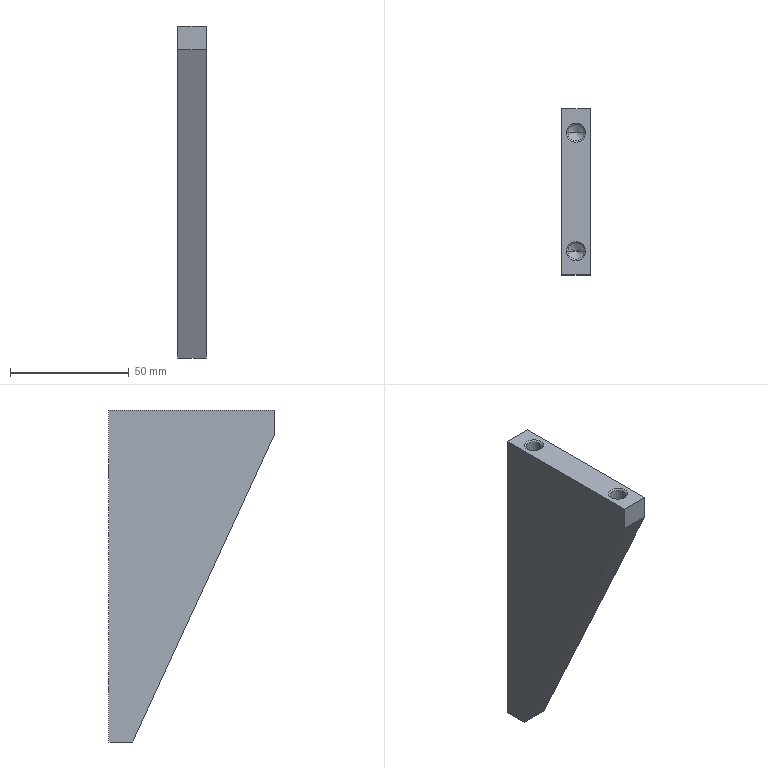Component | SolidWorks | DoubleFilmTransport-1_FilmPullingFixingBaseSupportPlate-2 | 1 solid | 31 faces | box 12 x 70 x 140 mm | volume 68032 mm3 | cone 16 | cylinder 8 | plane 7 | commonest cylinder face diameters 6.8 x8
build123d program:
from build123d import *

# Parameters (mm, degrees)
BOSS_EXTRUDE1_DEPTH            = 12
F_6_8_6_8_DIAMETER_HOLE1_D     = 6.8
F_6_8_6_8_DIAMETER_HOLE1_DEPTH = 18.25
F_6_8_6_8_DIAMETER_HOLE1_TIP   = 2.043
F_6_8_6_8_DIAMETER_HOLE2_D     = 6.8
F_6_8_6_8_DIAMETER_HOLE2_DEPTH = 18.25
F_6_8_6_8_DIAMETER_HOLE2_TIP   = 2.043
CHAMFER1_SIZE                  = 0.625


with BuildPart() as part:
    # Sketch1 → Boss-Extrude1 (new body)
    with BuildSketch(Plane(origin=(0, 0, -6), x_dir=(-1, 0, 0), z_dir=(0, 0, -1))):
        Polygon((0, 0), (0, 140), (-10, 140), (-70, 10), (-70, 0), align=None)
    extrude(amount=-BOSS_EXTRUDE1_DEPTH)

    # 6.8 _6.8_ Diameter Hole1
    with Locations(Plane.ZY):
        with Locations((0, 115), (0, 25)):
            Hole(F_6_8_6_8_DIAMETER_HOLE1_D / 2, depth=F_6_8_6_8_DIAMETER_HOLE1_DEPTH)
            with Locations((0, 0, -(F_6_8_6_8_DIAMETER_HOLE1_DEPTH + F_6_8_6_8_DIAMETER_HOLE1_TIP / 2))):  # 118° drill point
                Cone(0, F_6_8_6_8_DIAMETER_HOLE1_D / 2, F_6_8_6_8_DIAMETER_HOLE1_TIP, mode=Mode.SUBTRACT)

    # 6.8 _6.8_ Diameter Hole2
    with Locations(Plane(origin=(0, 0, 0), x_dir=(-1, 0, 0), z_dir=(0, -1, 0))):
        with Locations((-60, 0), (-10, 0)):
            Hole(F_6_8_6_8_DIAMETER_HOLE2_D / 2, depth=F_6_8_6_8_DIAMETER_HOLE2_DEPTH)
            with Locations((0, 0, -(F_6_8_6_8_DIAMETER_HOLE2_DEPTH + F_6_8_6_8_DIAMETER_HOLE2_TIP / 2))):  # 118° drill point
                Cone(0, F_6_8_6_8_DIAMETER_HOLE2_D / 2, F_6_8_6_8_DIAMETER_HOLE2_TIP, mode=Mode.SUBTRACT)

    # Chamfer1
    chamfer1_edges = [part.edges().sort_by_distance(p)[0] for p in [
        (0, 25, 3.4),
        (0, 115, 3.4),
        (6.6, 0, 0),
        (56.6, 0, 0),
    ]]
    chamfer(chamfer1_edges, length=CHAMFER1_SIZE)


solid = part.part

# Placed as in the assembly
solid = solid.moved(Location((-438.746, 33.373, -31.5), (-90, 90, 0)))
STEP:
#1=COLOUR_RGB('',0.7922,0.8196,0.9333);
#2=FILL_AREA_STYLE_COLOUR('',#1);
#3=FILL_AREA_STYLE('',(#2));
#4=SURFACE_STYLE_FILL_AREA(#3);
#5=SURFACE_SIDE_STYLE('',(#4));
#6=SURFACE_STYLE_USAGE(.BOTH.,#5);
#7=PRESENTATION_STYLE_ASSIGNMENT((#6));
#8=CARTESIAN_POINT('',(-17.14,0.9202,-1.265));
#9=VERTEX_POINT('',#8);
#10=CARTESIAN_POINT('',(-17.407,0.9202,-1.265));
#11=VERTEX_POINT('',#10);
#12=CARTESIAN_POINT('',(-17.273,0.9202,-1.265));
#13=DIRECTION('',(0.,0.,1.));
#14=DIRECTION('',(-1.,0.,0.));
#15=AXIS2_PLACEMENT_3D('',#12,#13,#14);
#16=CIRCLE('',#15,0.1339);
#17=EDGE_CURVE('',#9,#11,#16,.T.);
#18=ORIENTED_EDGE('',*,*,#17,.F.);
#19=CARTESIAN_POINT('',(-17.115,0.9202,-1.24));
#20=VERTEX_POINT('',#19);
#21=CARTESIAN_POINT('',(-17.14,0.9202,-1.265));
#22=DIRECTION('',(0.7071,0.,0.7071));
#23=VECTOR('',#22,39.37);
#24=LINE('',#21,#23);
#25=EDGE_CURVE('',#9,#20,#24,.T.);
#26=ORIENTED_EDGE('',*,*,#25,.T.);
#27=CARTESIAN_POINT('',(-17.432,0.9202,-1.24));
#28=VERTEX_POINT('',#27);
#29=CARTESIAN_POINT('',(-17.273,0.9202,-1.24));
#30=DIRECTION('',(-0.,0.,-1.));
#31=DIRECTION('',(0.,-1.,0.));
#32=AXIS2_PLACEMENT_3D('',#29,#30,#31);
#33=CIRCLE('',#32,0.1585);
#34=EDGE_CURVE('',#28,#20,#33,.T.);
#35=ORIENTED_EDGE('',*,*,#34,.F.);
#36=CARTESIAN_POINT('',(-17.407,0.9202,-1.265));
#37=DIRECTION('',(-0.7071,-0.,0.7071));
#38=VECTOR('',#37,39.37);
#39=LINE('',#36,#38);
#40=EDGE_CURVE('',#11,#28,#39,.T.);
#41=ORIENTED_EDGE('',*,*,#40,.F.);
#42=EDGE_LOOP('',(#18,#26,#35,#41));
#43=FACE_OUTER_BOUND('',#42,.T.);
#44=CARTESIAN_POINT('',(-17.273,0.9202,-1.265));
#45=DIRECTION('',(0.,0.,1.));
#46=DIRECTION('',(-1.,0.,0.));
#47=AXIS2_PLACEMENT_3D('',#44,#45,#46);
#48=CONICAL_SURFACE('',#47,0.1339,0.7854);
#49=ADVANCED_FACE('',(#43),#48,.F.);
#50=CARTESIAN_POINT('',(-17.14,-1.048,-1.265));
#51=VERTEX_POINT('',#50);
#52=CARTESIAN_POINT('',(-17.407,-1.048,-1.265));
#53=VERTEX_POINT('',#52);
#54=CARTESIAN_POINT('',(-17.273,-1.048,-1.265));
#55=DIRECTION('',(0.,0.,1.));
#56=DIRECTION('',(-1.,0.,0.));
#57=AXIS2_PLACEMENT_3D('',#54,#55,#56);
#58=CIRCLE('',#57,0.1339);
#59=EDGE_CURVE('',#51,#53,#58,.T.);
#60=ORIENTED_EDGE('',*,*,#59,.F.);
#61=CARTESIAN_POINT('',(-17.115,-1.048,-1.24));
#62=VERTEX_POINT('',#61);
#63=CARTESIAN_POINT('',(-17.14,-1.048,-1.265));
#64=DIRECTION('',(0.7071,0.,0.7071));
#65=VECTOR('',#64,39.37);
#66=LINE('',#63,#65);
#67=EDGE_CURVE('',#51,#62,#66,.T.);
#68=ORIENTED_EDGE('',*,*,#67,.T.);
#69=CARTESIAN_POINT('',(-17.432,-1.048,-1.24));
#70=VERTEX_POINT('',#69);
#71=CARTESIAN_POINT('',(-17.273,-1.048,-1.24));
#72=DIRECTION('',(-0.,0.,-1.));
#73=DIRECTION('',(0.,-1.,0.));
#74=AXIS2_PLACEMENT_3D('',#71,#72,#73);
#75=CIRCLE('',#74,0.1585);
#76=EDGE_CURVE('',#70,#62,#75,.T.);
#77=ORIENTED_EDGE('',*,*,#76,.F.);
#78=CARTESIAN_POINT('',(-17.407,-1.048,-1.265));
#79=DIRECTION('',(-0.7071,-0.,0.7071));
#80=VECTOR('',#79,39.37);
#81=LINE('',#78,#80);
#82=EDGE_CURVE('',#53,#70,#81,.T.);
#83=ORIENTED_EDGE('',*,*,#82,.F.);
#84=EDGE_LOOP('',(#60,#68,#77,#83));
#85=FACE_OUTER_BOUND('',#84,.T.);
#86=CARTESIAN_POINT('',(-17.273,-1.048,-1.265));
#87=DIRECTION('',(0.,0.,1.));
#88=DIRECTION('',(-1.,0.,0.));
#89=AXIS2_PLACEMENT_3D('',#86,#87,#88);
#90=CONICAL_SURFACE('',#89,0.1339,0.7854);
#91=ADVANCED_FACE('',(#85),#90,.F.);
#92=CARTESIAN_POINT('',(-17.407,1.289,-5.768));
#93=VERTEX_POINT('',#92);
#94=CARTESIAN_POINT('',(-17.14,1.289,-5.768));
#95=VERTEX_POINT('',#94);
#96=CARTESIAN_POINT('',(-17.273,1.289,-5.768));
#97=DIRECTION('',(-0.,1.,0.));
#98=DIRECTION('',(1.,0.,0.));
#99=AXIS2_PLACEMENT_3D('',#96,#97,#98);
#100=CIRCLE('',#99,0.1339);
#101=EDGE_CURVE('',#93,#95,#100,.T.);
#102=ORIENTED_EDGE('',*,*,#101,.F.);
#103=CARTESIAN_POINT('',(-17.432,1.314,-5.768));
#104=VERTEX_POINT('',#103);
#105=CARTESIAN_POINT('',(-17.407,1.289,-5.768));
#106=DIRECTION('',(-0.7071,0.7071,-0.));
#107=VECTOR('',#106,39.37);
#108=LINE('',#105,#107);
#109=EDGE_CURVE('',#93,#104,#108,.T.);
#110=ORIENTED_EDGE('',*,*,#109,.T.);
#111=CARTESIAN_POINT('',(-17.115,1.314,-5.768));
#112=VERTEX_POINT('',#111);
#113=CARTESIAN_POINT('',(-17.273,1.314,-5.768));
#114=DIRECTION('',(0.,-1.,0.));
#115=DIRECTION('',(1.,0.,0.));
#116=AXIS2_PLACEMENT_3D('',#113,#114,#115);
#117=CIRCLE('',#116,0.1585);
#118=EDGE_CURVE('',#112,#104,#117,.T.);
#119=ORIENTED_EDGE('',*,*,#118,.F.);
#120=CARTESIAN_POINT('',(-17.14,1.289,-5.768));
#121=DIRECTION('',(0.7071,0.7071,0.));
#122=VECTOR('',#121,39.37);
#123=LINE('',#120,#122);
#124=EDGE_CURVE('',#95,#112,#123,.T.);
#125=ORIENTED_EDGE('',*,*,#124,.F.);
#126=EDGE_LOOP('',(#102,#110,#119,#125));
#127=FACE_OUTER_BOUND('',#126,.T.);
#128=CARTESIAN_POINT('',(-17.273,1.289,-5.768));
#129=DIRECTION('',(-0.,1.,0.));
#130=DIRECTION('',(1.,0.,0.));
#131=AXIS2_PLACEMENT_3D('',#128,#129,#130);
#132=CONICAL_SURFACE('',#131,0.1339,0.7854);
#133=ADVANCED_FACE('',(#127),#132,.F.);
#134=CARTESIAN_POINT('',(-17.407,1.289,-2.224));
#135=VERTEX_POINT('',#134);
#136=CARTESIAN_POINT('',(-17.14,1.289,-2.224));
#137=VERTEX_POINT('',#136);
#138=CARTESIAN_POINT('',(-17.273,1.289,-2.224));
#139=DIRECTION('',(-0.,1.,0.));
#140=DIRECTION('',(1.,0.,0.));
#141=AXIS2_PLACEMENT_3D('',#138,#139,#140);
#142=CIRCLE('',#141,0.1339);
#143=EDGE_CURVE('',#135,#137,#142,.T.);
#144=ORIENTED_EDGE('',*,*,#143,.F.);
#145=CARTESIAN_POINT('',(-17.432,1.314,-2.224));
#146=VERTEX_POINT('',#145);
#147=CARTESIAN_POINT('',(-17.407,1.289,-2.224));
#148=DIRECTION('',(-0.7071,0.7071,-0.));
#149=VECTOR('',#148,39.37);
#150=LINE('',#147,#149);
#151=EDGE_CURVE('',#135,#146,#150,.T.);
#152=ORIENTED_EDGE('',*,*,#151,.T.);
#153=CARTESIAN_POINT('',(-17.115,1.314,-2.224));
#154=VERTEX_POINT('',#153);
#155=CARTESIAN_POINT('',(-17.273,1.314,-2.224));
#156=DIRECTION('',(0.,-1.,0.));
#157=DIRECTION('',(1.,0.,0.));
#158=AXIS2_PLACEMENT_3D('',#155,#156,#157);
#159=CIRCLE('',#158,0.1585);
#160=EDGE_CURVE('',#154,#146,#159,.T.);
#161=ORIENTED_EDGE('',*,*,#160,.F.);
#162=CARTESIAN_POINT('',(-17.14,1.289,-2.224));
#163=DIRECTION('',(0.7071,0.7071,0.));
#164=VECTOR('',#163,39.37);
#165=LINE('',#162,#164);
#166=EDGE_CURVE('',#137,#154,#165,.T.);
#167=ORIENTED_EDGE('',*,*,#166,.F.);
#168=EDGE_LOOP('',(#144,#152,#161,#167));
#169=FACE_OUTER_BOUND('',#168,.T.);
#170=CARTESIAN_POINT('',(-17.273,1.289,-2.224));
#171=DIRECTION('',(-0.,1.,0.));
#172=DIRECTION('',(1.,0.,0.));
#173=AXIS2_PLACEMENT_3D('',#170,#171,#172);
#174=CONICAL_SURFACE('',#173,0.1339,0.7854);
#175=ADVANCED_FACE('',(#169),#174,.F.);
#176=CARTESIAN_POINT('',(-17.14,-1.048,-1.959));
#177=VERTEX_POINT('',#176);
#178=CARTESIAN_POINT('',(-17.407,-1.048,-1.959));
#179=VERTEX_POINT('',#178);
#180=CARTESIAN_POINT('',(-17.273,-1.048,-1.959));
#181=DIRECTION('',(0.,0.,1.));
#182=DIRECTION('',(-1.,0.,0.));
#183=AXIS2_PLACEMENT_3D('',#180,#181,#182);
#184=CIRCLE('',#183,0.1339);
#185=EDGE_CURVE('',#177,#179,#184,.T.);
#186=ORIENTED_EDGE('',*,*,#185,.F.);
#187=CARTESIAN_POINT('',(-17.14,-1.048,-1.24));
#188=DIRECTION('',(0.,0.,1.));
#189=VECTOR('',#188,39.37);
#190=LINE('',#187,#189);
#191=EDGE_CURVE('',#177,#51,#190,.T.);
#192=ORIENTED_EDGE('',*,*,#191,.T.);
#193=ORIENTED_EDGE('',*,*,#59,.T.);
#194=CARTESIAN_POINT('',(-17.407,-1.048,-1.24));
#195=DIRECTION('',(0.,0.,1.));
#196=VECTOR('',#195,39.37);
#197=LINE('',#194,#196);
#198=EDGE_CURVE('',#179,#53,#197,.T.);
#199=ORIENTED_EDGE('',*,*,#198,.F.);
#200=EDGE_LOOP('',(#186,#192,#193,#199));
#201=FACE_OUTER_BOUND('',#200,.T.);
#202=CARTESIAN_POINT('',(-17.273,-1.048,-1.24));
#203=DIRECTION('',(0.,0.,1.));
#204=DIRECTION('',(-1.,0.,0.));
#205=AXIS2_PLACEMENT_3D('',#202,#203,#204);
#206=CYLINDRICAL_SURFACE('',#205,0.1339);
#207=ADVANCED_FACE('',(#201),#206,.F.);
#208=CARTESIAN_POINT('',(-17.273,-1.048,-2.039));
#209=VERTEX_POINT('',#208);
#210=CARTESIAN_POINT('',(-17.407,-1.048,-1.959));
#211=DIRECTION('',(-0.8572,-0.,0.515));
#212=VECTOR('',#211,39.37);
#213=LINE('',#210,#212);
#214=EDGE_CURVE('',#209,#179,#213,.T.);
#215=ORIENTED_EDGE('',*,*,#214,.F.);
#216=CARTESIAN_POINT('',(-17.14,-1.048,-1.959));
#217=DIRECTION('',(0.8572,0.,0.515));
#218=VECTOR('',#217,39.37);
#219=LINE('',#216,#218);
#220=EDGE_CURVE('',#209,#177,#219,.T.);
#221=ORIENTED_EDGE('',*,*,#220,.T.);
#222=ORIENTED_EDGE('',*,*,#185,.T.);
#223=EDGE_LOOP('',(#215,#221,#222));
#224=FACE_OUTER_BOUND('',#223,.T.);
#225=CARTESIAN_POINT('',(-17.273,-1.048,-1.959));
#226=DIRECTION('',(0.,0.,1.));
#227=DIRECTION('',(-1.,0.,0.));
#228=AXIS2_PLACEMENT_3D('',#225,#226,#227);
#229=CONICAL_SURFACE('',#228,0.1339,1.03);
#230=ADVANCED_FACE('',(#224),#229,.F.);
#231=CARTESIAN_POINT('',(-17.14,0.9202,-1.959));
#232=VERTEX_POINT('',#231);
#233=CARTESIAN_POINT('',(-17.407,0.9202,-1.959));
#234=VERTEX_POINT('',#233);
#235=CARTESIAN_POINT('',(-17.273,0.9202,-1.959));
#236=DIRECTION('',(0.,0.,1.));
#237=DIRECTION('',(-1.,0.,0.));
#238=AXIS2_PLACEMENT_3D('',#235,#236,#237);
#239=CIRCLE('',#238,0.1339);
#240=EDGE_CURVE('',#232,#234,#239,.T.);
#241=ORIENTED_EDGE('',*,*,#240,.F.);
#242=CARTESIAN_POINT('',(-17.14,0.9202,-1.24));
#243=DIRECTION('',(0.,0.,1.));
#244=VECTOR('',#243,39.37);
#245=LINE('',#242,#244);
#246=EDGE_CURVE('',#232,#9,#245,.T.);
#247=ORIENTED_EDGE('',*,*,#246,.T.);
#248=ORIENTED_EDGE('',*,*,#17,.T.);
#249=CARTESIAN_POINT('',(-17.407,0.9202,-1.24));
#250=DIRECTION('',(0.,0.,1.));
#251=VECTOR('',#250,39.37);
#252=LINE('',#249,#251);
#253=EDGE_CURVE('',#234,#11,#252,.T.);
#254=ORIENTED_EDGE('',*,*,#253,.F.);
#255=EDGE_LOOP('',(#241,#247,#248,#254));
#256=FACE_OUTER_BOUND('',#255,.T.);
#257=CARTESIAN_POINT('',(-17.273,0.9202,-1.24));
#258=DIRECTION('',(0.,0.,1.));
#259=DIRECTION('',(-1.,0.,0.));
#260=AXIS2_PLACEMENT_3D('',#257,#258,#259);
#261=CYLINDRICAL_SURFACE('',#260,0.1339);
#262=ADVANCED_FACE('',(#256),#261,.F.);
#263=CARTESIAN_POINT('',(-17.273,0.9202,-2.039));
#264=VERTEX_POINT('',#263);
#265=CARTESIAN_POINT('',(-17.407,0.9202,-1.959));
#266=DIRECTION('',(-0.8572,-0.,0.515));
#267=VECTOR('',#266,39.37);
#268=LINE('',#265,#267);
#269=EDGE_CURVE('',#264,#234,#268,.T.);
#270=ORIENTED_EDGE('',*,*,#269,.F.);
#271=CARTESIAN_POINT('',(-17.14,0.9202,-1.959));
#272=DIRECTION('',(0.8572,0.,0.515));
#273=VECTOR('',#272,39.37);
#274=LINE('',#271,#273);
#275=EDGE_CURVE('',#264,#232,#274,.T.);
#276=ORIENTED_EDGE('',*,*,#275,.T.);
#277=ORIENTED_EDGE('',*,*,#240,.T.);
#278=EDGE_LOOP('',(#270,#276,#277));
#279=FACE_OUTER_BOUND('',#278,.T.);
#280=CARTESIAN_POINT('',(-17.273,0.9202,-1.959));
#281=DIRECTION('',(0.,0.,1.));
#282=DIRECTION('',(-1.,0.,0.));
#283=AXIS2_PLACEMENT_3D('',#280,#281,#282);
#284=CONICAL_SURFACE('',#283,0.1339,1.03);
#285=ADVANCED_FACE('',(#279),#284,.F.);
#286=CARTESIAN_POINT('',(-17.407,0.5954,-5.768));
#287=VERTEX_POINT('',#286);
#288=CARTESIAN_POINT('',(-17.14,0.5954,-5.768));
#289=VERTEX_POINT('',#288);
#290=CARTESIAN_POINT('',(-17.273,0.5954,-5.768));
#291=DIRECTION('',(-0.,1.,0.));
#292=DIRECTION('',(1.,0.,0.));
#293=AXIS2_PLACEMENT_3D('',#290,#291,#292);
#294=CIRCLE('',#293,0.1339);
#295=EDGE_CURVE('',#287,#289,#294,.T.);
#296=ORIENTED_EDGE('',*,*,#295,.F.);
#297=CARTESIAN_POINT('',(-17.407,1.314,-5.768));
#298=DIRECTION('',(-0.,1.,0.));
#299=VECTOR('',#298,39.37);
#300=LINE('',#297,#299);
#301=EDGE_CURVE('',#287,#93,#300,.T.);
#302=ORIENTED_EDGE('',*,*,#301,.T.);
#303=ORIENTED_EDGE('',*,*,#101,.T.);
#304=CARTESIAN_POINT('',(-17.14,1.314,-5.768));
#305=DIRECTION('',(-0.,1.,0.));
#306=VECTOR('',#305,39.37);
#307=LINE('',#304,#306);
#308=EDGE_CURVE('',#289,#95,#307,.T.);
#309=ORIENTED_EDGE('',*,*,#308,.F.);
#310=EDGE_LOOP('',(#296,#302,#303,#309));
#311=FACE_OUTER_BOUND('',#310,.T.);
#312=CARTESIAN_POINT('',(-17.273,1.314,-5.768));
#313=DIRECTION('',(-0.,1.,0.));
#314=DIRECTION('',(1.,0.,0.));
#315=AXIS2_PLACEMENT_3D('',#312,#313,#314);
#316=CYLINDRICAL_SURFACE('',#315,0.1339);
#317=ADVANCED_FACE('',(#311),#316,.F.);
#318=CARTESIAN_POINT('',(-17.273,0.515,-5.768));
#319=VERTEX_POINT('',#318);
#320=CARTESIAN_POINT('',(-17.14,0.5954,-5.768));
#321=DIRECTION('',(0.8572,0.515,0.));
#322=VECTOR('',#321,39.37);
#323=LINE('',#320,#322);
#324=EDGE_CURVE('',#319,#289,#323,.T.);
#325=ORIENTED_EDGE('',*,*,#324,.F.);
#326=CARTESIAN_POINT('',(-17.407,0.5954,-5.768));
#327=DIRECTION('',(-0.8572,0.515,-0.));
#328=VECTOR('',#327,39.37);
#329=LINE('',#326,#328);
#330=EDGE_CURVE('',#319,#287,#329,.T.);
#331=ORIENTED_EDGE('',*,*,#330,.T.);
#332=ORIENTED_EDGE('',*,*,#295,.T.);
#333=EDGE_LOOP('',(#325,#331,#332));
#334=FACE_OUTER_BOUND('',#333,.T.);
#335=CARTESIAN_POINT('',(-17.273,0.5954,-5.768));
#336=DIRECTION('',(-0.,1.,0.));
#337=DIRECTION('',(1.,0.,0.));
#338=AXIS2_PLACEMENT_3D('',#335,#336,#337);
#339=CONICAL_SURFACE('',#338,0.1339,1.03);
#340=ADVANCED_FACE('',(#334),#339,.F.);
#341=CARTESIAN_POINT('',(-17.407,0.5954,-2.224));
#342=VERTEX_POINT('',#341);
#343=CARTESIAN_POINT('',(-17.14,0.5954,-2.224));
#344=VERTEX_POINT('',#343);
#345=CARTESIAN_POINT('',(-17.273,0.5954,-2.224));
#346=DIRECTION('',(-0.,1.,0.));
#347=DIRECTION('',(1.,0.,0.));
#348=AXIS2_PLACEMENT_3D('',#345,#346,#347);
#349=CIRCLE('',#348,0.1339);
#350=EDGE_CURVE('',#342,#344,#349,.T.);
#351=ORIENTED_EDGE('',*,*,#350,.F.);
#352=CARTESIAN_POINT('',(-17.407,1.314,-2.224));
#353=DIRECTION('',(-0.,1.,0.));
#354=VECTOR('',#353,39.37);
#355=LINE('',#352,#354);
#356=EDGE_CURVE('',#342,#135,#355,.T.);
#357=ORIENTED_EDGE('',*,*,#356,.T.);
#358=ORIENTED_EDGE('',*,*,#143,.T.);
#359=CARTESIAN_POINT('',(-17.14,1.314,-2.224));
#360=DIRECTION('',(-0.,1.,0.));
#361=VECTOR('',#360,39.37);
#362=LINE('',#359,#361);
#363=EDGE_CURVE('',#344,#137,#362,.T.);
#364=ORIENTED_EDGE('',*,*,#363,.F.);
#365=EDGE_LOOP('',(#351,#357,#358,#364));
#366=FACE_OUTER_BOUND('',#365,.T.);
#367=CARTESIAN_POINT('',(-17.273,1.314,-2.224));
#368=DIRECTION('',(-0.,1.,0.));
#369=DIRECTION('',(1.,0.,0.));
#370=AXIS2_PLACEMENT_3D('',#367,#368,#369);
#371=CYLINDRICAL_SURFACE('',#370,0.1339);
#372=ADVANCED_FACE('',(#366),#371,.F.);
#373=CARTESIAN_POINT('',(-17.273,0.515,-2.224));
#374=VERTEX_POINT('',#373);
#375=CARTESIAN_POINT('',(-17.14,0.5954,-2.224));
#376=DIRECTION('',(0.8572,0.515,0.));
#377=VECTOR('',#376,39.37);
#378=LINE('',#375,#377);
#379=EDGE_CURVE('',#374,#344,#378,.T.);
#380=ORIENTED_EDGE('',*,*,#379,.F.);
#381=CARTESIAN_POINT('',(-17.407,0.5954,-2.224));
#382=DIRECTION('',(-0.8572,0.515,-0.));
#383=VECTOR('',#382,39.37);
#384=LINE('',#381,#383);
#385=EDGE_CURVE('',#374,#342,#384,.T.);
#386=ORIENTED_EDGE('',*,*,#385,.T.);
#387=ORIENTED_EDGE('',*,*,#350,.T.);
#388=EDGE_LOOP('',(#380,#386,#387));
#389=FACE_OUTER_BOUND('',#388,.T.);
#390=CARTESIAN_POINT('',(-17.273,0.5954,-2.224));
#391=DIRECTION('',(-0.,1.,0.));
#392=DIRECTION('',(1.,0.,0.));
#393=AXIS2_PLACEMENT_3D('',#390,#391,#392);
#394=CONICAL_SURFACE('',#393,0.1339,1.03);
#395=ADVANCED_FACE('',(#389),#394,.F.);
#396=ORIENTED_EDGE('',*,*,#76,.T.);
#397=CARTESIAN_POINT('',(-17.273,-1.048,-1.24));
#398=DIRECTION('',(-0.,0.,-1.));
#399=DIRECTION('',(0.,-1.,0.));
#400=AXIS2_PLACEMENT_3D('',#397,#398,#399);
#401=CIRCLE('',#400,0.1585);
#402=EDGE_CURVE('',#62,#70,#401,.T.);
#403=ORIENTED_EDGE('',*,*,#402,.T.);
#404=EDGE_LOOP('',(#396,#403));
#405=FACE_BOUND('',#404,.T.);
#406=ORIENTED_EDGE('',*,*,#34,.T.);
#407=CARTESIAN_POINT('',(-17.273,0.9202,-1.24));
#408=DIRECTION('',(-0.,0.,-1.));
#409=DIRECTION('',(0.,-1.,0.));
#410=AXIS2_PLACEMENT_3D('',#407,#408,#409);
#411=CIRCLE('',#410,0.1585);
#412=EDGE_CURVE('',#20,#28,#411,.T.);
#413=ORIENTED_EDGE('',*,*,#412,.T.);
#414=EDGE_LOOP('',(#406,#413));
#415=FACE_BOUND('',#414,.T.);
#416=CARTESIAN_POINT('',(-17.51,-1.442,-1.24));
#417=VERTEX_POINT('',#416);
#418=CARTESIAN_POINT('',(-17.51,1.314,-1.24));
#419=VERTEX_POINT('',#418);
#420=CARTESIAN_POINT('',(-17.51,-1.442,-1.24));
#421=DIRECTION('',(-0.,1.,0.));
#422=VECTOR('',#421,39.37);
#423=LINE('',#420,#422);
#424=EDGE_CURVE('',#417,#419,#423,.T.);
#425=ORIENTED_EDGE('',*,*,#424,.F.);
#426=CARTESIAN_POINT('',(-17.037,-1.442,-1.24));
#427=VERTEX_POINT('',#426);
#428=CARTESIAN_POINT('',(-17.037,-1.442,-1.24));
#429=DIRECTION('',(-1.,-0.,0.));
#430=VECTOR('',#429,39.37);
#431=LINE('',#428,#430);
#432=EDGE_CURVE('',#427,#417,#431,.T.);
#433=ORIENTED_EDGE('',*,*,#432,.F.);
#434=CARTESIAN_POINT('',(-17.037,1.314,-1.24));
#435=VERTEX_POINT('',#434);
#436=CARTESIAN_POINT('',(-17.037,-1.442,-1.24));
#437=DIRECTION('',(-0.,1.,0.));
#438=VECTOR('',#437,39.37);
#439=LINE('',#436,#438);
#440=EDGE_CURVE('',#427,#435,#439,.T.);
#441=ORIENTED_EDGE('',*,*,#440,.T.);
#442=CARTESIAN_POINT('',(-17.037,1.314,-1.24));
#443=DIRECTION('',(-1.,-0.,0.));
#444=VECTOR('',#443,39.37);
#445=LINE('',#442,#444);
#446=EDGE_CURVE('',#435,#419,#445,.T.);
#447=ORIENTED_EDGE('',*,*,#446,.T.);
#448=EDGE_LOOP('',(#425,#433,#441,#447));
#449=FACE_OUTER_BOUND('',#448,.T.);
#450=CARTESIAN_POINT('',(-17.037,-1.442,-1.24));
#451=DIRECTION('',(0.,-0.,1.));
#452=DIRECTION('',(0.,-1.,-0.));
#453=AXIS2_PLACEMENT_3D('',#450,#451,#452);
#454=PLANE('',#453);
#455=ADVANCED_FACE('',(#405,#415,#449),#454,.T.);
#456=CARTESIAN_POINT('',(-17.51,-1.442,-1.634));
#457=VERTEX_POINT('',#456);
#458=CARTESIAN_POINT('',(-17.51,-1.442,-1.634));
#459=DIRECTION('',(0.,0.,1.));
#460=VECTOR('',#459,39.37);
#461=LINE('',#458,#460);
#462=EDGE_CURVE('',#457,#417,#461,.T.);
#463=ORIENTED_EDGE('',*,*,#462,.F.);
#464=CARTESIAN_POINT('',(-17.037,-1.442,-1.634));
#465=VERTEX_POINT('',#464);
#466=CARTESIAN_POINT('',(-17.037,-1.442,-1.634));
#467=DIRECTION('',(-1.,-0.,0.));
#468=VECTOR('',#467,39.37);
#469=LINE('',#466,#468);
#470=EDGE_CURVE('',#465,#457,#469,.T.);
#471=ORIENTED_EDGE('',*,*,#470,.F.);
#472=CARTESIAN_POINT('',(-17.037,-1.442,-1.634));
#473=DIRECTION('',(0.,0.,1.));
#474=VECTOR('',#473,39.37);
#475=LINE('',#472,#474);
#476=EDGE_CURVE('',#465,#427,#475,.T.);
#477=ORIENTED_EDGE('',*,*,#476,.T.);
#478=ORIENTED_EDGE('',*,*,#432,.T.);
#479=EDGE_LOOP('',(#463,#471,#477,#478));
#480=FACE_OUTER_BOUND('',#479,.T.);
#481=CARTESIAN_POINT('',(-17.037,-1.442,-1.634));
#482=DIRECTION('',(0.,-1.,0.));
#483=DIRECTION('',(-1.,-0.,0.));
#484=AXIS2_PLACEMENT_3D('',#481,#482,#483);
#485=PLANE('',#484);
#486=ADVANCED_FACE('',(#480),#485,.T.);
#487=CARTESIAN_POINT('',(-17.51,0.9202,-6.752));
#488=VERTEX_POINT('',#487);
#489=CARTESIAN_POINT('',(-17.51,0.9202,-6.752));
#490=DIRECTION('',(0.,-0.4191,0.908));
#491=VECTOR('',#490,39.37);
#492=LINE('',#489,#491);
#493=EDGE_CURVE('',#488,#457,#492,.T.);
#494=ORIENTED_EDGE('',*,*,#493,.F.);
#495=CARTESIAN_POINT('',(-17.037,0.9202,-6.752));
#496=VERTEX_POINT('',#495);
#497=CARTESIAN_POINT('',(-17.037,0.9202,-6.752));
#498=DIRECTION('',(-1.,-0.,0.));
#499=VECTOR('',#498,39.37);
#500=LINE('',#497,#499);
#501=EDGE_CURVE('',#496,#488,#500,.T.);
#502=ORIENTED_EDGE('',*,*,#501,.F.);
#503=CARTESIAN_POINT('',(-17.037,0.9202,-6.752));
#504=DIRECTION('',(0.,-0.4191,0.908));
#505=VECTOR('',#504,39.37);
#506=LINE('',#503,#505);
#507=EDGE_CURVE('',#496,#465,#506,.T.);
#508=ORIENTED_EDGE('',*,*,#507,.T.);
#509=ORIENTED_EDGE('',*,*,#470,.T.);
#510=EDGE_LOOP('',(#494,#502,#508,#509));
#511=FACE_OUTER_BOUND('',#510,.T.);
#512=CARTESIAN_POINT('',(-17.037,0.9202,-6.752));
#513=DIRECTION('',(0.,-0.908,-0.4191));
#514=DIRECTION('',(-0.,0.4191,-0.908));
#515=AXIS2_PLACEMENT_3D('',#512,#513,#514);
#516=PLANE('',#515);
#517=ADVANCED_FACE('',(#511),#516,.T.);
#518=CARTESIAN_POINT('',(-17.51,1.314,-6.752));
#519=VERTEX_POINT('',#518);
#520=CARTESIAN_POINT('',(-17.51,1.314,-6.752));
#521=DIRECTION('',(0.,-1.,0.));
#522=VECTOR('',#521,39.37);
#523=LINE('',#520,#522);
#524=EDGE_CURVE('',#519,#488,#523,.T.);
#525=ORIENTED_EDGE('',*,*,#524,.F.);
#526=CARTESIAN_POINT('',(-17.037,1.314,-6.752));
#527=VERTEX_POINT('',#526);
#528=CARTESIAN_POINT('',(-17.037,1.314,-6.752));
#529=DIRECTION('',(-1.,-0.,0.));
#530=VECTOR('',#529,39.37);
#531=LINE('',#528,#530);
#532=EDGE_CURVE('',#527,#519,#531,.T.);
#533=ORIENTED_EDGE('',*,*,#532,.F.);
#534=CARTESIAN_POINT('',(-17.037,1.314,-6.752));
#535=DIRECTION('',(0.,-1.,0.));
#536=VECTOR('',#535,39.37);
#537=LINE('',#534,#536);
#538=EDGE_CURVE('',#527,#496,#537,.T.);
#539=ORIENTED_EDGE('',*,*,#538,.T.);
#540=ORIENTED_EDGE('',*,*,#501,.T.);
#541=EDGE_LOOP('',(#525,#533,#539,#540));
#542=FACE_OUTER_BOUND('',#541,.T.);
#543=CARTESIAN_POINT('',(-17.037,1.314,-6.752));
#544=DIRECTION('',(0.,0.,-1.));
#545=DIRECTION('',(1.,0.,0.));
#546=AXIS2_PLACEMENT_3D('',#543,#544,#545);
#547=PLANE('',#546);
#548=ADVANCED_FACE('',(#542),#547,.T.);
#549=ORIENTED_EDGE('',*,*,#160,.T.);
#550=CARTESIAN_POINT('',(-17.273,1.314,-2.224));
#551=DIRECTION('',(0.,-1.,0.));
#552=DIRECTION('',(1.,0.,0.));
#553=AXIS2_PLACEMENT_3D('',#550,#551,#552);
#554=CIRCLE('',#553,0.1585);
#555=EDGE_CURVE('',#146,#154,#554,.T.);
#556=ORIENTED_EDGE('',*,*,#555,.T.);
#557=EDGE_LOOP('',(#549,#556));
#558=FACE_BOUND('',#557,.T.);
#559=ORIENTED_EDGE('',*,*,#118,.T.);
#560=CARTESIAN_POINT('',(-17.273,1.314,-5.768));
#561=DIRECTION('',(0.,-1.,0.));
#562=DIRECTION('',(1.,0.,0.));
#563=AXIS2_PLACEMENT_3D('',#560,#561,#562);
#564=CIRCLE('',#563,0.1585);
#565=EDGE_CURVE('',#104,#112,#564,.T.);
#566=ORIENTED_EDGE('',*,*,#565,.T.);
#567=EDGE_LOOP('',(#559,#566));
#568=FACE_BOUND('',#567,.T.);
#569=CARTESIAN_POINT('',(-17.51,1.314,-1.24));
#570=DIRECTION('',(0.,0.,-1.));
#571=VECTOR('',#570,39.37);
#572=LINE('',#569,#571);
#573=EDGE_CURVE('',#419,#519,#572,.T.);
#574=ORIENTED_EDGE('',*,*,#573,.F.);
#575=ORIENTED_EDGE('',*,*,#446,.F.);
#576=CARTESIAN_POINT('',(-17.037,1.314,-1.24));
#577=DIRECTION('',(0.,0.,-1.));
#578=VECTOR('',#577,39.37);
#579=LINE('',#576,#578);
#580=EDGE_CURVE('',#435,#527,#579,.T.);
#581=ORIENTED_EDGE('',*,*,#580,.T.);
#582=ORIENTED_EDGE('',*,*,#532,.T.);
#583=EDGE_LOOP('',(#574,#575,#581,#582));
#584=FACE_OUTER_BOUND('',#583,.T.);
#585=CARTESIAN_POINT('',(-17.037,1.314,-1.24));
#586=DIRECTION('',(-0.,1.,0.));
#587=DIRECTION('',(1.,0.,0.));
#588=AXIS2_PLACEMENT_3D('',#585,#586,#587);
#589=PLANE('',#588);
#590=ADVANCED_FACE('',(#558,#568,#584),#589,.T.);
#591=ORIENTED_EDGE('',*,*,#440,.F.);
#592=ORIENTED_EDGE('',*,*,#476,.F.);
#593=ORIENTED_EDGE('',*,*,#507,.F.);
#594=ORIENTED_EDGE('',*,*,#538,.F.);
#595=ORIENTED_EDGE('',*,*,#580,.F.);
#596=EDGE_LOOP('',(#591,#592,#593,#594,#595));
#597=FACE_OUTER_BOUND('',#596,.T.);
#598=CARTESIAN_POINT('',(-17.037,1.314,-1.24));
#599=DIRECTION('',(-1.,-0.,0.));
#600=DIRECTION('',(-0.,1.,0.));
#601=AXIS2_PLACEMENT_3D('',#598,#599,#600);
#602=PLANE('',#601);
#603=ADVANCED_FACE('',(#597),#602,.F.);
#604=ORIENTED_EDGE('',*,*,#424,.T.);
#605=ORIENTED_EDGE('',*,*,#573,.T.);
#606=ORIENTED_EDGE('',*,*,#524,.T.);
#607=ORIENTED_EDGE('',*,*,#493,.T.);
#608=ORIENTED_EDGE('',*,*,#462,.T.);
#609=EDGE_LOOP('',(#604,#605,#606,#607,#608));
#610=FACE_OUTER_BOUND('',#609,.T.);
#611=CARTESIAN_POINT('',(-17.51,1.314,-1.24));
#612=DIRECTION('',(-1.,-0.,0.));
#613=DIRECTION('',(-0.,1.,0.));
#614=AXIS2_PLACEMENT_3D('',#611,#612,#613);
#615=PLANE('',#614);
#616=ADVANCED_FACE('',(#610),#615,.T.);
#617=ORIENTED_EDGE('',*,*,#385,.F.);
#618=ORIENTED_EDGE('',*,*,#379,.T.);
#619=CARTESIAN_POINT('',(-17.273,0.5954,-2.224));
#620=DIRECTION('',(-0.,1.,0.));
#621=DIRECTION('',(1.,0.,0.));
#622=AXIS2_PLACEMENT_3D('',#619,#620,#621);
#623=CIRCLE('',#622,0.1339);
#624=EDGE_CURVE('',#344,#342,#623,.T.);
#625=ORIENTED_EDGE('',*,*,#624,.T.);
#626=EDGE_LOOP('',(#617,#618,#625));
#627=FACE_OUTER_BOUND('',#626,.T.);
#628=CARTESIAN_POINT('',(-17.273,0.5954,-2.224));
#629=DIRECTION('',(-0.,1.,0.));
#630=DIRECTION('',(1.,0.,0.));
#631=AXIS2_PLACEMENT_3D('',#628,#629,#630);
#632=CONICAL_SURFACE('',#631,0.1339,1.03);
#633=ADVANCED_FACE('',(#627),#632,.F.);
#634=ORIENTED_EDGE('',*,*,#356,.F.);
#635=ORIENTED_EDGE('',*,*,#624,.F.);
#636=ORIENTED_EDGE('',*,*,#363,.T.);
#637=CARTESIAN_POINT('',(-17.273,1.289,-2.224));
#638=DIRECTION('',(-0.,1.,0.));
#639=DIRECTION('',(1.,0.,0.));
#640=AXIS2_PLACEMENT_3D('',#637,#638,#639);
#641=CIRCLE('',#640,0.1339);
#642=EDGE_CURVE('',#137,#135,#641,.T.);
#643=ORIENTED_EDGE('',*,*,#642,.T.);
#644=EDGE_LOOP('',(#634,#635,#636,#643));
#645=FACE_OUTER_BOUND('',#644,.T.);
#646=CARTESIAN_POINT('',(-17.273,1.314,-2.224));
#647=DIRECTION('',(-0.,1.,0.));
#648=DIRECTION('',(1.,0.,0.));
#649=AXIS2_PLACEMENT_3D('',#646,#647,#648);
#650=CYLINDRICAL_SURFACE('',#649,0.1339);
#651=ADVANCED_FACE('',(#645),#650,.F.);
#652=ORIENTED_EDGE('',*,*,#330,.F.);
#653=ORIENTED_EDGE('',*,*,#324,.T.);
#654=CARTESIAN_POINT('',(-17.273,0.5954,-5.768));
#655=DIRECTION('',(-0.,1.,0.));
#656=DIRECTION('',(1.,0.,0.));
#657=AXIS2_PLACEMENT_3D('',#654,#655,#656);
#658=CIRCLE('',#657,0.1339);
#659=EDGE_CURVE('',#289,#287,#658,.T.);
#660=ORIENTED_EDGE('',*,*,#659,.T.);
#661=EDGE_LOOP('',(#652,#653,#660));
#662=FACE_OUTER_BOUND('',#661,.T.);
#663=CARTESIAN_POINT('',(-17.273,0.5954,-5.768));
#664=DIRECTION('',(-0.,1.,0.));
#665=DIRECTION('',(1.,0.,0.));
#666=AXIS2_PLACEMENT_3D('',#663,#664,#665);
#667=CONICAL_SURFACE('',#666,0.1339,1.03);
#668=ADVANCED_FACE('',(#662),#667,.F.);
#669=ORIENTED_EDGE('',*,*,#301,.F.);
#670=ORIENTED_EDGE('',*,*,#659,.F.);
#671=ORIENTED_EDGE('',*,*,#308,.T.);
#672=CARTESIAN_POINT('',(-17.273,1.289,-5.768));
#673=DIRECTION('',(-0.,1.,0.));
#674=DIRECTION('',(1.,0.,0.));
#675=AXIS2_PLACEMENT_3D('',#672,#673,#674);
#676=CIRCLE('',#675,0.1339);
#677=EDGE_CURVE('',#95,#93,#676,.T.);
#678=ORIENTED_EDGE('',*,*,#677,.T.);
#679=EDGE_LOOP('',(#669,#670,#671,#678));
#680=FACE_OUTER_BOUND('',#679,.T.);
#681=CARTESIAN_POINT('',(-17.273,1.314,-5.768));
#682=DIRECTION('',(-0.,1.,0.));
#683=DIRECTION('',(1.,0.,0.));
#684=AXIS2_PLACEMENT_3D('',#681,#682,#683);
#685=CYLINDRICAL_SURFACE('',#684,0.1339);
#686=ADVANCED_FACE('',(#680),#685,.F.);
#687=ORIENTED_EDGE('',*,*,#275,.F.);
#688=ORIENTED_EDGE('',*,*,#269,.T.);
#689=CARTESIAN_POINT('',(-17.273,0.9202,-1.959));
#690=DIRECTION('',(0.,0.,1.));
#691=DIRECTION('',(-1.,0.,0.));
#692=AXIS2_PLACEMENT_3D('',#689,#690,#691);
#693=CIRCLE('',#692,0.1339);
#694=EDGE_CURVE('',#234,#232,#693,.T.);
#695=ORIENTED_EDGE('',*,*,#694,.T.);
#696=EDGE_LOOP('',(#687,#688,#695));
#697=FACE_OUTER_BOUND('',#696,.T.);
#698=CARTESIAN_POINT('',(-17.273,0.9202,-1.959));
#699=DIRECTION('',(0.,0.,1.));
#700=DIRECTION('',(-1.,0.,0.));
#701=AXIS2_PLACEMENT_3D('',#698,#699,#700);
#702=CONICAL_SURFACE('',#701,0.1339,1.03);
#703=ADVANCED_FACE('',(#697),#702,.F.);
#704=ORIENTED_EDGE('',*,*,#246,.F.);
#705=ORIENTED_EDGE('',*,*,#694,.F.);
#706=ORIENTED_EDGE('',*,*,#253,.T.);
#707=CARTESIAN_POINT('',(-17.273,0.9202,-1.265));
#708=DIRECTION('',(0.,0.,1.));
#709=DIRECTION('',(-1.,0.,0.));
#710=AXIS2_PLACEMENT_3D('',#707,#708,#709);
#711=CIRCLE('',#710,0.1339);
#712=EDGE_CURVE('',#11,#9,#711,.T.);
#713=ORIENTED_EDGE('',*,*,#712,.T.);
#714=EDGE_LOOP('',(#704,#705,#706,#713));
#715=FACE_OUTER_BOUND('',#714,.T.);
#716=CARTESIAN_POINT('',(-17.273,0.9202,-1.24));
#717=DIRECTION('',(0.,0.,1.));
#718=DIRECTION('',(-1.,0.,0.));
#719=AXIS2_PLACEMENT_3D('',#716,#717,#718);
#720=CYLINDRICAL_SURFACE('',#719,0.1339);
#721=ADVANCED_FACE('',(#715),#720,.F.);
#722=ORIENTED_EDGE('',*,*,#220,.F.);
#723=ORIENTED_EDGE('',*,*,#214,.T.);
#724=CARTESIAN_POINT('',(-17.273,-1.048,-1.959));
#725=DIRECTION('',(0.,0.,1.));
#726=DIRECTION('',(-1.,0.,0.));
#727=AXIS2_PLACEMENT_3D('',#724,#725,#726);
#728=CIRCLE('',#727,0.1339);
#729=EDGE_CURVE('',#179,#177,#728,.T.);
#730=ORIENTED_EDGE('',*,*,#729,.T.);
#731=EDGE_LOOP('',(#722,#723,#730));
#732=FACE_OUTER_BOUND('',#731,.T.);
#733=CARTESIAN_POINT('',(-17.273,-1.048,-1.959));
#734=DIRECTION('',(0.,0.,1.));
#735=DIRECTION('',(-1.,0.,0.));
#736=AXIS2_PLACEMENT_3D('',#733,#734,#735);
#737=CONICAL_SURFACE('',#736,0.1339,1.03);
#738=ADVANCED_FACE('',(#732),#737,.F.);
#739=ORIENTED_EDGE('',*,*,#191,.F.);
#740=ORIENTED_EDGE('',*,*,#729,.F.);
#741=ORIENTED_EDGE('',*,*,#198,.T.);
#742=CARTESIAN_POINT('',(-17.273,-1.048,-1.265));
#743=DIRECTION('',(0.,0.,1.));
#744=DIRECTION('',(-1.,0.,0.));
#745=AXIS2_PLACEMENT_3D('',#742,#743,#744);
#746=CIRCLE('',#745,0.1339);
#747=EDGE_CURVE('',#53,#51,#746,.T.);
#748=ORIENTED_EDGE('',*,*,#747,.T.);
#749=EDGE_LOOP('',(#739,#740,#741,#748));
#750=FACE_OUTER_BOUND('',#749,.T.);
#751=CARTESIAN_POINT('',(-17.273,-1.048,-1.24));
#752=DIRECTION('',(0.,0.,1.));
#753=DIRECTION('',(-1.,0.,0.));
#754=AXIS2_PLACEMENT_3D('',#751,#752,#753);
#755=CYLINDRICAL_SURFACE('',#754,0.1339);
#756=ADVANCED_FACE('',(#750),#755,.F.);
#757=ORIENTED_EDGE('',*,*,#151,.F.);
#758=ORIENTED_EDGE('',*,*,#642,.F.);
#759=ORIENTED_EDGE('',*,*,#166,.T.);
#760=ORIENTED_EDGE('',*,*,#555,.F.);
#761=EDGE_LOOP('',(#757,#758,#759,#760));
#762=FACE_OUTER_BOUND('',#761,.T.);
#763=CARTESIAN_POINT('',(-17.273,1.289,-2.224));
#764=DIRECTION('',(-0.,1.,0.));
#765=DIRECTION('',(1.,0.,0.));
#766=AXIS2_PLACEMENT_3D('',#763,#764,#765);
#767=CONICAL_SURFACE('',#766,0.1339,0.7854);
#768=ADVANCED_FACE('',(#762),#767,.F.);
#769=ORIENTED_EDGE('',*,*,#109,.F.);
#770=ORIENTED_EDGE('',*,*,#677,.F.);
#771=ORIENTED_EDGE('',*,*,#124,.T.);
#772=ORIENTED_EDGE('',*,*,#565,.F.);
#773=EDGE_LOOP('',(#769,#770,#771,#772));
#774=FACE_OUTER_BOUND('',#773,.T.);
#775=CARTESIAN_POINT('',(-17.273,1.289,-5.768));
#776=DIRECTION('',(-0.,1.,0.));
#777=DIRECTION('',(1.,0.,0.));
#778=AXIS2_PLACEMENT_3D('',#775,#776,#777);
#779=CONICAL_SURFACE('',#778,0.1339,0.7854);
#780=ADVANCED_FACE('',(#774),#779,.F.);
#781=ORIENTED_EDGE('',*,*,#67,.F.);
#782=ORIENTED_EDGE('',*,*,#747,.F.);
#783=ORIENTED_EDGE('',*,*,#82,.T.);
#784=ORIENTED_EDGE('',*,*,#402,.F.);
#785=EDGE_LOOP('',(#781,#782,#783,#784));
#786=FACE_OUTER_BOUND('',#785,.T.);
#787=CARTESIAN_POINT('',(-17.273,-1.048,-1.265));
#788=DIRECTION('',(0.,0.,1.));
#789=DIRECTION('',(-1.,0.,0.));
#790=AXIS2_PLACEMENT_3D('',#787,#788,#789);
#791=CONICAL_SURFACE('',#790,0.1339,0.7854);
#792=ADVANCED_FACE('',(#786),#791,.F.);
#793=ORIENTED_EDGE('',*,*,#25,.F.);
#794=ORIENTED_EDGE('',*,*,#712,.F.);
#795=ORIENTED_EDGE('',*,*,#40,.T.);
#796=ORIENTED_EDGE('',*,*,#412,.F.);
#797=EDGE_LOOP('',(#793,#794,#795,#796));
#798=FACE_OUTER_BOUND('',#797,.T.);
#799=CARTESIAN_POINT('',(-17.273,0.9202,-1.265));
#800=DIRECTION('',(0.,0.,1.));
#801=DIRECTION('',(-1.,0.,0.));
#802=AXIS2_PLACEMENT_3D('',#799,#800,#801);
#803=CONICAL_SURFACE('',#802,0.1339,0.7854);
#804=ADVANCED_FACE('',(#798),#803,.F.);
#805=CLOSED_SHELL('',(#49,#91,#133,#175,#207,#230,#262,#285,#317,#340,#372,#395,#455,#486,#517,#548,#590,#603,#616,#633,#651,#668,#686,#703,#721,#738,#756,#768,#780,#792,#804));
#806=MANIFOLD_SOLID_BREP('',#805);
#807=STYLED_ITEM('',(#7),#806);
#808=(LENGTH_UNIT()NAMED_UNIT(*)SI_UNIT($,.METRE.));
#809=LENGTH_MEASURE_WITH_UNIT(LENGTH_MEASURE(0.0254),#808);
#810=DIMENSIONAL_EXPONENTS(1.,0.,0.,0.,0.,0.,0.);
#811=(CONVERSION_BASED_UNIT('',#809)LENGTH_UNIT()NAMED_UNIT(#810));
#812=UNCERTAINTY_MEASURE_WITH_UNIT(LENGTH_MEASURE(0.00001),#811,'','');
#813=(NAMED_UNIT(*)PLANE_ANGLE_UNIT()SI_UNIT($,.RADIAN.));
#814=(NAMED_UNIT(*)SI_UNIT($,.STERADIAN.)SOLID_ANGLE_UNIT());
#815=(GEOMETRIC_REPRESENTATION_CONTEXT(3)GLOBAL_UNCERTAINTY_ASSIGNED_CONTEXT((#812))GLOBAL_UNIT_ASSIGNED_CONTEXT((#811,#813,#814))REPRESENTATION_CONTEXT('',''));
#816=MECHANICAL_DESIGN_GEOMETRIC_PRESENTATION_REPRESENTATION('',(#807),#815);
#817=CARTESIAN_POINT('',(0.,0.,0.));
#818=DIRECTION('',(0.,0.,1.));
#819=DIRECTION('',(1.,0.,0.));
#820=AXIS2_PLACEMENT_3D('',#817,#818,#819);
#821=(LENGTH_UNIT()NAMED_UNIT(*)SI_UNIT($,.METRE.));
#822=LENGTH_MEASURE_WITH_UNIT(LENGTH_MEASURE(0.0254),#821);
#823=DIMENSIONAL_EXPONENTS(1.,0.,0.,0.,0.,0.,0.);
#824=(CONVERSION_BASED_UNIT('',#822)LENGTH_UNIT()NAMED_UNIT(#823));
#825=UNCERTAINTY_MEASURE_WITH_UNIT(LENGTH_MEASURE(0.00001),#824,'','');
#826=(NAMED_UNIT(*)PLANE_ANGLE_UNIT()SI_UNIT($,.RADIAN.));
#827=(NAMED_UNIT(*)SI_UNIT($,.STERADIAN.)SOLID_ANGLE_UNIT());
#828=(GEOMETRIC_REPRESENTATION_CONTEXT(3)GLOBAL_UNCERTAINTY_ASSIGNED_CONTEXT((#825))GLOBAL_UNIT_ASSIGNED_CONTEXT((#824,#826,#827))REPRESENTATION_CONTEXT('',''));
#829=ADVANCED_BREP_SHAPE_REPRESENTATION('',(#806,#820),#828);
#830=PRESENTATION_LAYER_ASSIGNMENT('','',(#807));